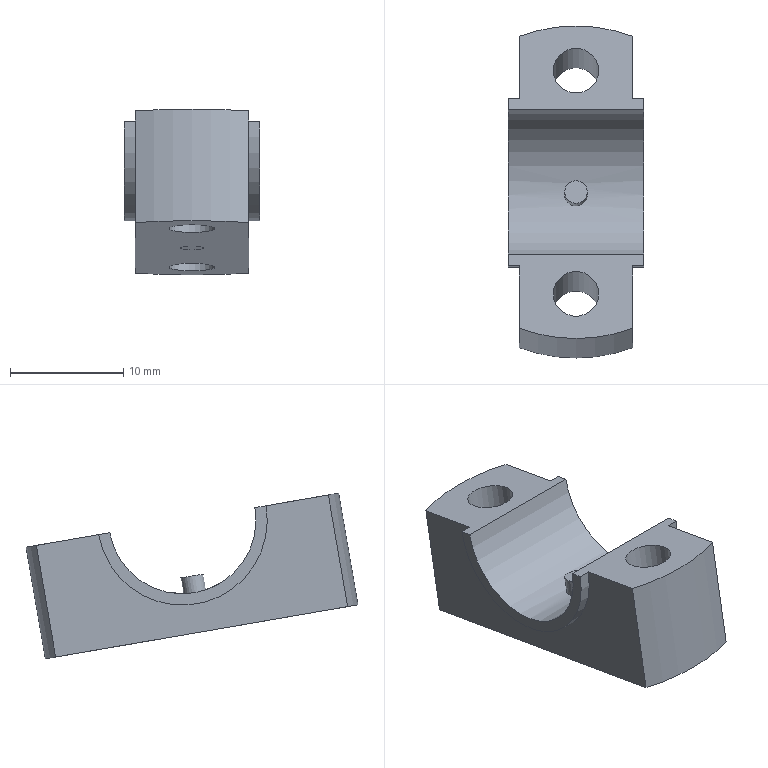Component | NX | 17B__27_2 | 2 solids | 18 faces | volume 1873 mm3 | cylinder 9 | plane 9 | commonest cylinder face diameters 28 x2 15 x2 2 x2 4 x2 13 x1